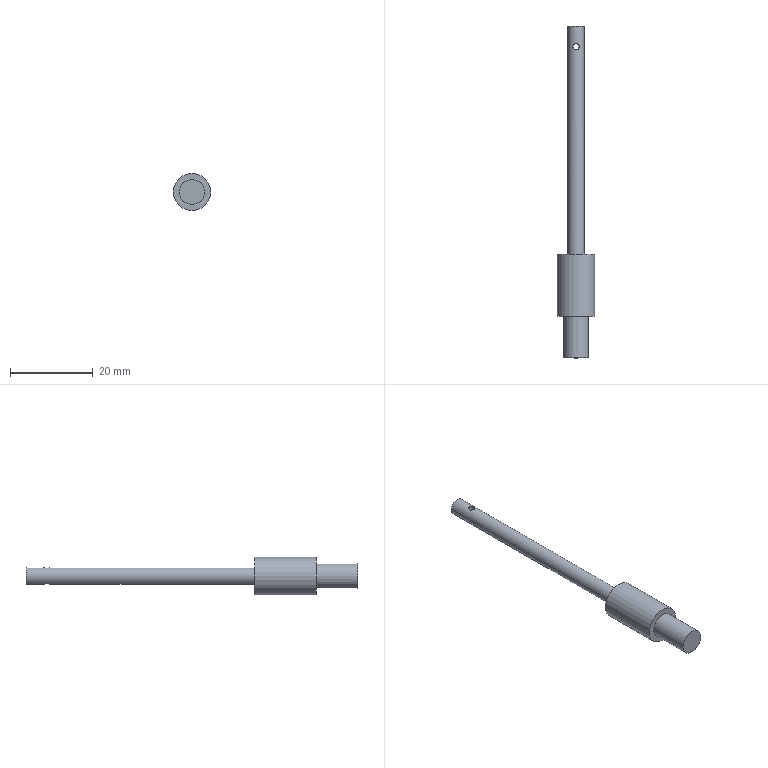Component | NX | PIN | 1 solid | 8 faces | box 9 x 80 x 9 mm | volume 1921 mm3 | cylinder 4 | plane 4 | commonest cylinder face diameters 6 x1 9 x1 4 x1 1.5 x1
STEP:
#1=CARTESIAN_POINT('',(0.,0.,0.));
#2=DIRECTION('',(0.,0.,1.));
#3=DIRECTION('',(1.,0.,0.));
#4=AXIS2_PLACEMENT_3D('',#1,#2,#3);
#5=CARTESIAN_POINT('',(-3.,0.,33.5));
#6=VERTEX_POINT('',#5);
#7=CARTESIAN_POINT('',(0.,0.,33.5));
#8=DIRECTION('',(0.,1.,0.));
#9=DIRECTION('',(-1.,0.,0.));
#10=AXIS2_PLACEMENT_3D('',#7,#8,#9);
#11=CIRCLE('',#10,3.);
#12=CARTESIAN_POINT('',(0.,0.,33.5));
#13=DIRECTION('',(0.,-1.,0.));
#14=DIRECTION('',(0.,0.,1.));
#15=AXIS2_PLACEMENT_3D('',#12,#13,#14);
#16=CYLINDRICAL_SURFACE('',#15,3.);
#17=CARTESIAN_POINT('',(7.854,0.));
#18=DIRECTION('',(-1.,0.));
#19=VECTOR('',#18,1.);
#20=LINE('',#17,#19);
#21=(GEOMETRIC_REPRESENTATION_CONTEXT(2)PARAMETRIC_REPRESENTATION_CONTEXT()REPRESENTATION_CONTEXT('',''));
#22=DEFINITIONAL_REPRESENTATION('',(#20),#21);
#23=PCURVE('',#16,#22);
#24=CARTESIAN_POINT('',(0.,0.,33.5));
#25=DIRECTION('',(0.,1.,0.));
#26=DIRECTION('',(0.,0.,-1.));
#27=AXIS2_PLACEMENT_3D('',#24,#25,#26);
#28=PLANE('',#27);
#29=CARTESIAN_POINT('',(0.,0.));
#30=DIRECTION('',(0.,1.));
#31=AXIS2_PLACEMENT_2D('',#29,#30);
#32=CIRCLE('',#31,3.);
#33=(GEOMETRIC_REPRESENTATION_CONTEXT(2)PARAMETRIC_REPRESENTATION_CONTEXT()REPRESENTATION_CONTEXT('',''));
#34=DEFINITIONAL_REPRESENTATION('',(#32),#33);
#35=PCURVE('',#28,#34);
#36=SURFACE_CURVE('',#11,(#23,#35),.PCURVE_S1.);
#37=EDGE_CURVE('',#6,#6,#36,.T.);
#38=ORIENTED_EDGE('',*,*,#37,.F.);
#39=CARTESIAN_POINT('',(-3.,-10.,33.5));
#40=VERTEX_POINT('',#39);
#41=CARTESIAN_POINT('',(-3.,0.,33.5));
#42=CARTESIAN_POINT('',(-3.,-10.,33.5));
#43=B_SPLINE_CURVE_WITH_KNOTS('',1,(#41,#42),.UNSPECIFIED.,.F.,.F.,(2,2),(0.,10.),.PIECEWISE_BEZIER_KNOTS.);
#44=CARTESIAN_POINT('',(7.854,0.));
#45=DIRECTION('',(0.,1.));
#46=VECTOR('',#45,1.);
#47=LINE('',#44,#46);
#48=(GEOMETRIC_REPRESENTATION_CONTEXT(2)PARAMETRIC_REPRESENTATION_CONTEXT()REPRESENTATION_CONTEXT('',''));
#49=DEFINITIONAL_REPRESENTATION('',(#47),#48);
#50=PCURVE('',#16,#49);
#51=CARTESIAN_POINT('',(1.571,0.));
#52=DIRECTION('',(0.,1.));
#53=VECTOR('',#52,1.);
#54=LINE('',#51,#53);
#55=(GEOMETRIC_REPRESENTATION_CONTEXT(2)PARAMETRIC_REPRESENTATION_CONTEXT()REPRESENTATION_CONTEXT('',''));
#56=DEFINITIONAL_REPRESENTATION('',(#54),#55);
#57=PCURVE('',#16,#56);
#58=SEAM_CURVE('',#43,(#50,#57),.PCURVE_S1.);
#59=EDGE_CURVE('',#6,#40,#58,.T.);
#60=ORIENTED_EDGE('',*,*,#59,.T.);
#61=CARTESIAN_POINT('',(0.,-10.,33.5));
#62=DIRECTION('',(0.,1.,0.));
#63=DIRECTION('',(-1.,0.,0.));
#64=AXIS2_PLACEMENT_3D('',#61,#62,#63);
#65=CIRCLE('',#64,3.);
#66=CARTESIAN_POINT('',(7.854,10.));
#67=DIRECTION('',(-1.,0.));
#68=VECTOR('',#67,1.);
#69=LINE('',#66,#68);
#70=(GEOMETRIC_REPRESENTATION_CONTEXT(2)PARAMETRIC_REPRESENTATION_CONTEXT()REPRESENTATION_CONTEXT('',''));
#71=DEFINITIONAL_REPRESENTATION('',(#69),#70);
#72=PCURVE('',#16,#71);
#73=CARTESIAN_POINT('',(0.,-10.,33.5));
#74=DIRECTION('',(0.,1.,0.));
#75=DIRECTION('',(0.,0.,-1.));
#76=AXIS2_PLACEMENT_3D('',#73,#74,#75);
#77=PLANE('',#76);
#78=CARTESIAN_POINT('',(0.,0.));
#79=DIRECTION('',(0.,1.));
#80=AXIS2_PLACEMENT_2D('',#78,#79);
#81=CIRCLE('',#80,3.);
#82=(GEOMETRIC_REPRESENTATION_CONTEXT(2)PARAMETRIC_REPRESENTATION_CONTEXT()REPRESENTATION_CONTEXT('',''));
#83=DEFINITIONAL_REPRESENTATION('',(#81),#82);
#84=PCURVE('',#77,#83);
#85=SURFACE_CURVE('',#65,(#72,#84),.PCURVE_S1.);
#86=EDGE_CURVE('',#40,#40,#85,.T.);
#87=ORIENTED_EDGE('',*,*,#86,.T.);
#88=ORIENTED_EDGE('',*,*,#59,.F.);
#89=EDGE_LOOP('',(#38,#60,#87,#88));
#90=FACE_BOUND('',#89,.T.);
#91=ADVANCED_FACE('',(#90),#16,.T.);
#92=ORIENTED_EDGE('',*,*,#86,.F.);
#93=EDGE_LOOP('',(#92));
#94=FACE_BOUND('',#93,.T.);
#95=ADVANCED_FACE('',(#94),#77,.F.);
#96=CARTESIAN_POINT('',(-4.5,15.,33.5));
#97=VERTEX_POINT('',#96);
#98=CARTESIAN_POINT('',(0.,15.,33.5));
#99=DIRECTION('',(0.,1.,0.));
#100=DIRECTION('',(-1.,0.,0.));
#101=AXIS2_PLACEMENT_3D('',#98,#99,#100);
#102=CIRCLE('',#101,4.5);
#103=CARTESIAN_POINT('',(0.,15.,33.5));
#104=DIRECTION('',(0.,-1.,0.));
#105=DIRECTION('',(0.,0.,1.));
#106=AXIS2_PLACEMENT_3D('',#103,#104,#105);
#107=CYLINDRICAL_SURFACE('',#106,4.5);
#108=CARTESIAN_POINT('',(7.854,0.));
#109=DIRECTION('',(-1.,0.));
#110=VECTOR('',#109,1.);
#111=LINE('',#108,#110);
#112=(GEOMETRIC_REPRESENTATION_CONTEXT(2)PARAMETRIC_REPRESENTATION_CONTEXT()REPRESENTATION_CONTEXT('',''));
#113=DEFINITIONAL_REPRESENTATION('',(#111),#112);
#114=PCURVE('',#107,#113);
#115=CARTESIAN_POINT('',(0.,15.,33.5));
#116=DIRECTION('',(0.,1.,0.));
#117=DIRECTION('',(0.,0.,-1.));
#118=AXIS2_PLACEMENT_3D('',#115,#116,#117);
#119=PLANE('',#118);
#120=CARTESIAN_POINT('',(0.,0.));
#121=DIRECTION('',(0.,1.));
#122=AXIS2_PLACEMENT_2D('',#120,#121);
#123=CIRCLE('',#122,4.5);
#124=(GEOMETRIC_REPRESENTATION_CONTEXT(2)PARAMETRIC_REPRESENTATION_CONTEXT()REPRESENTATION_CONTEXT('',''));
#125=DEFINITIONAL_REPRESENTATION('',(#123),#124);
#126=PCURVE('',#119,#125);
#127=SURFACE_CURVE('',#102,(#114,#126),.PCURVE_S1.);
#128=EDGE_CURVE('',#97,#97,#127,.T.);
#129=ORIENTED_EDGE('',*,*,#128,.F.);
#130=CARTESIAN_POINT('',(-4.5,0.,33.5));
#131=VERTEX_POINT('',#130);
#132=CARTESIAN_POINT('',(-4.5,15.,33.5));
#133=CARTESIAN_POINT('',(-4.5,0.,33.5));
#134=B_SPLINE_CURVE_WITH_KNOTS('',1,(#132,#133),.UNSPECIFIED.,.F.,.F.,(2,2),(0.,15.),.PIECEWISE_BEZIER_KNOTS.);
#135=CARTESIAN_POINT('',(7.854,0.));
#136=DIRECTION('',(0.,1.));
#137=VECTOR('',#136,1.);
#138=LINE('',#135,#137);
#139=(GEOMETRIC_REPRESENTATION_CONTEXT(2)PARAMETRIC_REPRESENTATION_CONTEXT()REPRESENTATION_CONTEXT('',''));
#140=DEFINITIONAL_REPRESENTATION('',(#138),#139);
#141=PCURVE('',#107,#140);
#142=CARTESIAN_POINT('',(1.571,0.));
#143=DIRECTION('',(0.,1.));
#144=VECTOR('',#143,1.);
#145=LINE('',#142,#144);
#146=(GEOMETRIC_REPRESENTATION_CONTEXT(2)PARAMETRIC_REPRESENTATION_CONTEXT()REPRESENTATION_CONTEXT('',''));
#147=DEFINITIONAL_REPRESENTATION('',(#145),#146);
#148=PCURVE('',#107,#147);
#149=SEAM_CURVE('',#134,(#141,#148),.PCURVE_S1.);
#150=EDGE_CURVE('',#97,#131,#149,.T.);
#151=ORIENTED_EDGE('',*,*,#150,.T.);
#152=CARTESIAN_POINT('',(0.,0.,33.5));
#153=DIRECTION('',(0.,1.,0.));
#154=DIRECTION('',(-1.,0.,0.));
#155=AXIS2_PLACEMENT_3D('',#152,#153,#154);
#156=CIRCLE('',#155,4.5);
#157=CARTESIAN_POINT('',(7.854,15.));
#158=DIRECTION('',(-1.,0.));
#159=VECTOR('',#158,1.);
#160=LINE('',#157,#159);
#161=(GEOMETRIC_REPRESENTATION_CONTEXT(2)PARAMETRIC_REPRESENTATION_CONTEXT()REPRESENTATION_CONTEXT('',''));
#162=DEFINITIONAL_REPRESENTATION('',(#160),#161);
#163=PCURVE('',#107,#162);
#164=CARTESIAN_POINT('',(0.,0.));
#165=DIRECTION('',(0.,1.));
#166=AXIS2_PLACEMENT_2D('',#164,#165);
#167=CIRCLE('',#166,4.5);
#168=(GEOMETRIC_REPRESENTATION_CONTEXT(2)PARAMETRIC_REPRESENTATION_CONTEXT()REPRESENTATION_CONTEXT('',''));
#169=DEFINITIONAL_REPRESENTATION('',(#167),#168);
#170=PCURVE('',#28,#169);
#171=SURFACE_CURVE('',#156,(#163,#170),.PCURVE_S1.);
#172=EDGE_CURVE('',#131,#131,#171,.T.);
#173=ORIENTED_EDGE('',*,*,#172,.T.);
#174=ORIENTED_EDGE('',*,*,#150,.F.);
#175=EDGE_LOOP('',(#129,#151,#173,#174));
#176=FACE_BOUND('',#175,.T.);
#177=ADVANCED_FACE('',(#176),#107,.T.);
#178=CARTESIAN_POINT('',(-2.,15.,33.5));
#179=VERTEX_POINT('',#178);
#180=CARTESIAN_POINT('',(0.,15.,33.5));
#181=DIRECTION('',(0.,1.,0.));
#182=DIRECTION('',(-1.,0.,0.));
#183=AXIS2_PLACEMENT_3D('',#180,#181,#182);
#184=CIRCLE('',#183,2.);
#185=CARTESIAN_POINT('',(0.,0.));
#186=DIRECTION('',(0.,1.));
#187=AXIS2_PLACEMENT_2D('',#185,#186);
#188=CIRCLE('',#187,2.);
#189=(GEOMETRIC_REPRESENTATION_CONTEXT(2)PARAMETRIC_REPRESENTATION_CONTEXT()REPRESENTATION_CONTEXT('',''));
#190=DEFINITIONAL_REPRESENTATION('',(#188),#189);
#191=PCURVE('',#119,#190);
#192=CARTESIAN_POINT('',(0.,70.,33.5));
#193=DIRECTION('',(0.,-1.,0.));
#194=DIRECTION('',(0.,0.,1.));
#195=AXIS2_PLACEMENT_3D('',#192,#193,#194);
#196=CYLINDRICAL_SURFACE('',#195,2.);
#197=CARTESIAN_POINT('',(7.854,55.));
#198=DIRECTION('',(-1.,0.));
#199=VECTOR('',#198,1.);
#200=LINE('',#197,#199);
#201=(GEOMETRIC_REPRESENTATION_CONTEXT(2)PARAMETRIC_REPRESENTATION_CONTEXT()REPRESENTATION_CONTEXT('',''));
#202=DEFINITIONAL_REPRESENTATION('',(#200),#201);
#203=PCURVE('',#196,#202);
#204=SURFACE_CURVE('',#184,(#191,#203),.PCURVE_S1.);
#205=EDGE_CURVE('',#179,#179,#204,.T.);
#206=ORIENTED_EDGE('',*,*,#205,.F.);
#207=EDGE_LOOP('',(#206));
#208=FACE_BOUND('',#207,.T.);
#209=ORIENTED_EDGE('',*,*,#128,.T.);
#210=EDGE_LOOP('',(#209));
#211=FACE_BOUND('',#210,.T.);
#212=ADVANCED_FACE('',(#208,#211),#119,.T.);
#213=ORIENTED_EDGE('',*,*,#37,.T.);
#214=EDGE_LOOP('',(#213));
#215=FACE_BOUND('',#214,.T.);
#216=ORIENTED_EDGE('',*,*,#172,.F.);
#217=EDGE_LOOP('',(#216));
#218=FACE_BOUND('',#217,.T.);
#219=ADVANCED_FACE('',(#215,#218),#28,.F.);
#220=CARTESIAN_POINT('',(-2.,70.,33.5));
#221=VERTEX_POINT('',#220);
#222=CARTESIAN_POINT('',(0.,70.,33.5));
#223=DIRECTION('',(0.,1.,0.));
#224=DIRECTION('',(-1.,0.,0.));
#225=AXIS2_PLACEMENT_3D('',#222,#223,#224);
#226=CIRCLE('',#225,2.);
#227=CARTESIAN_POINT('',(7.854,0.));
#228=DIRECTION('',(-1.,0.));
#229=VECTOR('',#228,1.);
#230=LINE('',#227,#229);
#231=(GEOMETRIC_REPRESENTATION_CONTEXT(2)PARAMETRIC_REPRESENTATION_CONTEXT()REPRESENTATION_CONTEXT('',''));
#232=DEFINITIONAL_REPRESENTATION('',(#230),#231);
#233=PCURVE('',#196,#232);
#234=CARTESIAN_POINT('',(0.,70.,33.5));
#235=DIRECTION('',(0.,1.,0.));
#236=DIRECTION('',(0.,0.,-1.));
#237=AXIS2_PLACEMENT_3D('',#234,#235,#236);
#238=PLANE('',#237);
#239=CARTESIAN_POINT('',(0.,0.));
#240=DIRECTION('',(0.,1.));
#241=AXIS2_PLACEMENT_2D('',#239,#240);
#242=CIRCLE('',#241,2.);
#243=(GEOMETRIC_REPRESENTATION_CONTEXT(2)PARAMETRIC_REPRESENTATION_CONTEXT()REPRESENTATION_CONTEXT('',''));
#244=DEFINITIONAL_REPRESENTATION('',(#242),#243);
#245=PCURVE('',#238,#244);
#246=SURFACE_CURVE('',#226,(#233,#245),.PCURVE_S1.);
#247=EDGE_CURVE('',#221,#221,#246,.T.);
#248=ORIENTED_EDGE('',*,*,#247,.F.);
#249=CARTESIAN_POINT('',(-2.,70.,33.5));
#250=CARTESIAN_POINT('',(-2.,15.,33.5));
#251=B_SPLINE_CURVE_WITH_KNOTS('',1,(#249,#250),.UNSPECIFIED.,.F.,.F.,(2,2),(0.,55.),.PIECEWISE_BEZIER_KNOTS.);
#252=CARTESIAN_POINT('',(7.854,0.));
#253=DIRECTION('',(0.,1.));
#254=VECTOR('',#253,1.);
#255=LINE('',#252,#254);
#256=(GEOMETRIC_REPRESENTATION_CONTEXT(2)PARAMETRIC_REPRESENTATION_CONTEXT()REPRESENTATION_CONTEXT('',''));
#257=DEFINITIONAL_REPRESENTATION('',(#255),#256);
#258=PCURVE('',#196,#257);
#259=CARTESIAN_POINT('',(1.571,0.));
#260=DIRECTION('',(0.,1.));
#261=VECTOR('',#260,1.);
#262=LINE('',#259,#261);
#263=(GEOMETRIC_REPRESENTATION_CONTEXT(2)PARAMETRIC_REPRESENTATION_CONTEXT()REPRESENTATION_CONTEXT('',''));
#264=DEFINITIONAL_REPRESENTATION('',(#262),#263);
#265=PCURVE('',#196,#264);
#266=SEAM_CURVE('',#251,(#258,#265),.PCURVE_S1.);
#267=EDGE_CURVE('',#221,#179,#266,.T.);
#268=ORIENTED_EDGE('',*,*,#267,.T.);
#269=ORIENTED_EDGE('',*,*,#205,.T.);
#270=ORIENTED_EDGE('',*,*,#267,.F.);
#271=EDGE_LOOP('',(#248,#268,#269,#270));
#272=FACE_BOUND('',#271,.T.);
#273=CARTESIAN_POINT('',(0.,65.75,35.5));
#274=VERTEX_POINT('',#273);
#275=CARTESIAN_POINT('',(0.,65.75,35.5));
#276=CARTESIAN_POINT('',(0.08082,65.75,35.5));
#277=CARTESIAN_POINT('',(0.1627,65.737,35.495));
#278=CARTESIAN_POINT('',(0.2389,65.711,35.486));
#279=CARTESIAN_POINT('',(0.3149,65.685,35.477));
#280=CARTESIAN_POINT('',(0.3872,65.647,35.463));
#281=CARTESIAN_POINT('',(0.4506,65.6,35.449));
#282=CARTESIAN_POINT('',(0.5165,65.55,35.433));
#283=CARTESIAN_POINT('',(0.5746,65.489,35.416));
#284=CARTESIAN_POINT('',(0.6209,65.421,35.401));
#285=CARTESIAN_POINT('',(0.6689,65.35,35.386));
#286=CARTESIAN_POINT('',(0.7053,65.269,35.372));
#287=CARTESIAN_POINT('',(0.7267,65.185,35.363));
#288=CARTESIAN_POINT('',(0.7472,65.105,35.355));
#289=CARTESIAN_POINT('',(0.7544,65.019,35.352));
#290=CARTESIAN_POINT('',(0.7473,64.936,35.355));
#291=CARTESIAN_POINT('',(0.7406,64.858,35.358));
#292=CARTESIAN_POINT('',(0.7213,64.78,35.366));
#293=CARTESIAN_POINT('',(0.6912,64.709,35.377));
#294=CARTESIAN_POINT('',(0.6605,64.636,35.388));
#295=CARTESIAN_POINT('',(0.6179,64.568,35.403));
#296=CARTESIAN_POINT('',(0.5665,64.508,35.418));
#297=CARTESIAN_POINT('',(0.5116,64.445,35.434));
#298=CARTESIAN_POINT('',(0.4452,64.391,35.451));
#299=CARTESIAN_POINT('',(0.3721,64.349,35.465));
#300=CARTESIAN_POINT('',(0.298,64.306,35.479));
#301=CARTESIAN_POINT('',(0.2147,64.276,35.49));
#302=CARTESIAN_POINT('',(0.1297,64.261,35.496));
#303=CARTESIAN_POINT('',(0.04914,64.247,35.501));
#304=CARTESIAN_POINT('',(-0.03529,64.246,35.501));
#305=CARTESIAN_POINT('',(-0.1161,64.259,35.497));
#306=CARTESIAN_POINT('',(-0.1938,64.271,35.492));
#307=CARTESIAN_POINT('',(-0.2703,64.296,35.483));
#308=CARTESIAN_POINT('',(-0.3397,64.331,35.471));
#309=CARTESIAN_POINT('',(-0.4112,64.368,35.459));
#310=CARTESIAN_POINT('',(-0.4772,64.416,35.443));
#311=CARTESIAN_POINT('',(-0.5332,64.473,35.428));
#312=CARTESIAN_POINT('',(-0.5925,64.533,35.411));
#313=CARTESIAN_POINT('',(-0.6423,64.604,35.394));
#314=CARTESIAN_POINT('',(-0.6784,64.68,35.381));
#315=CARTESIAN_POINT('',(-0.7147,64.757,35.368));
#316=CARTESIAN_POINT('',(-0.7383,64.843,35.359));
#317=CARTESIAN_POINT('',(-0.7466,64.928,35.355));
#318=CARTESIAN_POINT('',(-0.7543,65.008,35.352));
#319=CARTESIAN_POINT('',(-0.7488,65.091,35.355));
#320=CARTESIAN_POINT('',(-0.7306,65.169,35.362));
#321=CARTESIAN_POINT('',(-0.713,65.245,35.369));
#322=CARTESIAN_POINT('',(-0.6832,65.319,35.38));
#323=CARTESIAN_POINT('',(-0.6437,65.385,35.394));
#324=CARTESIAN_POINT('',(-0.602,65.455,35.408));
#325=CARTESIAN_POINT('',(-0.5486,65.518,35.424));
#326=CARTESIAN_POINT('',(-0.4871,65.57,35.44));
#327=CARTESIAN_POINT('',(-0.4223,65.626,35.456));
#328=CARTESIAN_POINT('',(-0.3467,65.671,35.471));
#329=CARTESIAN_POINT('',(-0.2662,65.701,35.482));
#330=CARTESIAN_POINT('',(-0.1823,65.733,35.493));
#331=CARTESIAN_POINT('',(-0.09041,65.75,35.5));
#332=CARTESIAN_POINT('',(0.,65.75,35.5));
#333=B_SPLINE_CURVE_WITH_KNOTS('',3,(#275,#276,#277,#278,#279,#280,#281,#282,#283,#284,#285,#286,#287,#288,#289,#290,#291,#292,#293,#294,#295,#296,#297,#298,#299,#300,#301,#302,#303,#304,#305,#306,#307,#308,#309,#310,#311,#312,#313,#314,#315,#316,#317,#318,#319,#320,#321,#322,#323,#324,#325,#326,#327,#328,#329,#330,#331,#332),.UNSPECIFIED.,.T.,.F.,(1,3,3,3,3,3,3,3,3,3,3,3,3,3,3,3,3,3,3,3,3,1),(-0.05748,0.,0.05123,0.1023,0.1554,0.2106,0.2635,0.3131,0.3637,0.4177,0.4726,0.5246,0.5744,0.6258,0.6802,0.7349,0.786,0.8354,0.8875,0.9425,1.,1.051),.UNSPECIFIED.);
#334=CARTESIAN_POINT('',(6.283,4.25));
#335=CARTESIAN_POINT('',(6.274,4.25));
#336=CARTESIAN_POINT('',(6.256,4.251));
#337=CARTESIAN_POINT('',(6.229,4.257));
#338=CARTESIAN_POINT('',(6.203,4.267));
#339=CARTESIAN_POINT('',(6.176,4.28));
#340=CARTESIAN_POINT('',(6.151,4.297));
#341=CARTESIAN_POINT('',(6.126,4.318));
#342=CARTESIAN_POINT('',(6.102,4.342));
#343=CARTESIAN_POINT('',(6.078,4.369));
#344=CARTESIAN_POINT('',(6.056,4.4));
#345=CARTESIAN_POINT('',(6.035,4.433));
#346=CARTESIAN_POINT('',(6.015,4.469));
#347=CARTESIAN_POINT('',(5.996,4.508));
#348=CARTESIAN_POINT('',(5.978,4.55));
#349=CARTESIAN_POINT('',(5.962,4.593));
#350=CARTESIAN_POINT('',(5.948,4.639));
#351=CARTESIAN_POINT('',(5.935,4.687));
#352=CARTESIAN_POINT('',(5.924,4.736));
#353=CARTESIAN_POINT('',(5.915,4.787));
#354=CARTESIAN_POINT('',(5.908,4.839));
#355=CARTESIAN_POINT('',(5.903,4.892));
#356=CARTESIAN_POINT('',(5.9,4.946));
#357=CARTESIAN_POINT('',(5.898,5.));
#358=CARTESIAN_POINT('',(5.899,5.054));
#359=CARTESIAN_POINT('',(5.903,5.107));
#360=CARTESIAN_POINT('',(5.908,5.161));
#361=CARTESIAN_POINT('',(5.915,5.213));
#362=CARTESIAN_POINT('',(5.924,5.264));
#363=CARTESIAN_POINT('',(5.935,5.313));
#364=CARTESIAN_POINT('',(5.948,5.361));
#365=CARTESIAN_POINT('',(5.962,5.407));
#366=CARTESIAN_POINT('',(5.978,5.451));
#367=CARTESIAN_POINT('',(5.996,5.492));
#368=CARTESIAN_POINT('',(6.015,5.531));
#369=CARTESIAN_POINT('',(6.035,5.567));
#370=CARTESIAN_POINT('',(6.056,5.6));
#371=CARTESIAN_POINT('',(6.078,5.631));
#372=CARTESIAN_POINT('',(6.102,5.658));
#373=CARTESIAN_POINT('',(6.126,5.682));
#374=CARTESIAN_POINT('',(6.151,5.703));
#375=CARTESIAN_POINT('',(6.176,5.72));
#376=CARTESIAN_POINT('',(6.203,5.733));
#377=CARTESIAN_POINT('',(6.229,5.743));
#378=CARTESIAN_POINT('',(6.256,5.749));
#379=CARTESIAN_POINT('',(6.283,5.751));
#380=CARTESIAN_POINT('',(6.31,5.749));
#381=CARTESIAN_POINT('',(6.337,5.743));
#382=CARTESIAN_POINT('',(6.364,5.733));
#383=CARTESIAN_POINT('',(6.39,5.72));
#384=CARTESIAN_POINT('',(6.416,5.703));
#385=CARTESIAN_POINT('',(6.441,5.682));
#386=CARTESIAN_POINT('',(6.465,5.658));
#387=CARTESIAN_POINT('',(6.488,5.631));
#388=CARTESIAN_POINT('',(6.511,5.6));
#389=CARTESIAN_POINT('',(6.532,5.567));
#390=CARTESIAN_POINT('',(6.552,5.53));
#391=CARTESIAN_POINT('',(6.571,5.492));
#392=CARTESIAN_POINT('',(6.588,5.45));
#393=CARTESIAN_POINT('',(6.604,5.407));
#394=CARTESIAN_POINT('',(6.619,5.361));
#395=CARTESIAN_POINT('',(6.631,5.313));
#396=CARTESIAN_POINT('',(6.642,5.264));
#397=CARTESIAN_POINT('',(6.651,5.213));
#398=CARTESIAN_POINT('',(6.659,5.161));
#399=CARTESIAN_POINT('',(6.664,5.108));
#400=CARTESIAN_POINT('',(6.667,5.054));
#401=CARTESIAN_POINT('',(6.668,5.));
#402=CARTESIAN_POINT('',(6.667,4.946));
#403=CARTESIAN_POINT('',(6.664,4.892));
#404=CARTESIAN_POINT('',(6.659,4.839));
#405=CARTESIAN_POINT('',(6.651,4.787));
#406=CARTESIAN_POINT('',(6.642,4.736));
#407=CARTESIAN_POINT('',(6.631,4.686));
#408=CARTESIAN_POINT('',(6.618,4.639));
#409=CARTESIAN_POINT('',(6.604,4.593));
#410=CARTESIAN_POINT('',(6.588,4.549));
#411=CARTESIAN_POINT('',(6.57,4.508));
#412=CARTESIAN_POINT('',(6.552,4.469));
#413=CARTESIAN_POINT('',(6.532,4.433));
#414=CARTESIAN_POINT('',(6.51,4.4));
#415=CARTESIAN_POINT('',(6.488,4.369));
#416=CARTESIAN_POINT('',(6.464,4.342));
#417=CARTESIAN_POINT('',(6.44,4.318));
#418=CARTESIAN_POINT('',(6.415,4.297));
#419=CARTESIAN_POINT('',(6.39,4.28));
#420=CARTESIAN_POINT('',(6.364,4.267));
#421=CARTESIAN_POINT('',(6.337,4.257));
#422=CARTESIAN_POINT('',(6.31,4.251));
#423=CARTESIAN_POINT('',(6.292,4.25));
#424=CARTESIAN_POINT('',(6.283,4.25));
#425=B_SPLINE_CURVE_WITH_KNOTS('',3,(#334,#335,#336,#337,#338,#339,#340,#341,#342,#343,#344,#345,#346,#347,#348,#349,#350,#351,#352,#353,#354,#355,#356,#357,#358,#359,#360,#361,#362,#363,#364,#365,#366,#367,#368,#369,#370,#371,#372,#373,#374,#375,#376,#377,#378,#379,#380,#381,#382,#383,#384,#385,#386,#387,#388,#389,#390,#391,#392,#393,#394,#395,#396,#397,#398,#399,#400,#401,#402,#403,#404,#405,#406,#407,#408,#409,#410,#411,#412,#413,#414,#415,#416,#417,#418,#419,#420,#421,#422,#423,#424),.UNSPECIFIED.,.T.,.F.,(4,1,1,1,1,1,1,1,1,1,1,1,1,1,1,1,1,1,1,1,1,1,1,1,1,1,1,1,1,1,1,1,1,1,1,1,1,1,1,1,1,1,1,1,1,1,1,1,1,1,1,1,1,1,1,1,1,1,1,1,1,1,1,1,1,1,1,1,1,1,1,1,1,1,1,1,1,1,1,1,1,1,1,1,1,1,1,1,4),(0.,0.01136,0.02273,0.03409,0.04545,0.05682,0.06818,0.07955,0.09091,0.1023,0.1136,0.125,0.1364,0.1477,0.1591,0.1705,0.1818,0.1932,0.2045,0.2159,0.2273,0.2386,0.25,0.2614,0.2727,0.2841,0.2955,0.3068,0.3182,0.3295,0.3409,0.3523,0.3636,0.375,0.3864,0.3977,0.4091,0.4205,0.4318,0.4432,0.4545,0.4659,0.4773,0.4886,0.5,0.5114,0.5227,0.5341,0.5455,0.5568,0.5682,0.5795,0.5909,0.6023,0.6136,0.625,0.6364,0.6477,0.6591,0.6705,0.6818,0.6932,0.7045,0.7159,0.7273,0.7386,0.75,0.7614,0.7727,0.7841,0.7955,0.8068,0.8182,0.8295,0.8409,0.8523,0.8636,0.875,0.8864,0.8977,0.9091,0.9205,0.9318,0.9432,0.9545,0.9659,0.9773,0.9886,1.),.QUASI_UNIFORM_KNOTS.);
#426=(GEOMETRIC_REPRESENTATION_CONTEXT(2)PARAMETRIC_REPRESENTATION_CONTEXT()REPRESENTATION_CONTEXT('',''));
#427=DEFINITIONAL_REPRESENTATION('',(#425),#426);
#428=PCURVE('',#196,#427);
#429=CARTESIAN_POINT('',(0.,65.,15.5));
#430=DIRECTION('',(0.,0.,1.));
#431=DIRECTION('',(0.,1.,0.));
#432=AXIS2_PLACEMENT_3D('',#429,#430,#431);
#433=CYLINDRICAL_SURFACE('',#432,0.75);
#434=CARTESIAN_POINT('',(6.283,20.));
#435=CARTESIAN_POINT('',(6.259,20.));
#436=CARTESIAN_POINT('',(6.211,19.999));
#437=CARTESIAN_POINT('',(6.139,19.997));
#438=CARTESIAN_POINT('',(6.067,19.994));
#439=CARTESIAN_POINT('',(5.995,19.989));
#440=CARTESIAN_POINT('',(5.924,19.983));
#441=CARTESIAN_POINT('',(5.852,19.975));
#442=CARTESIAN_POINT('',(5.781,19.967));
#443=CARTESIAN_POINT('',(5.71,19.958));
#444=CARTESIAN_POINT('',(5.639,19.949));
#445=CARTESIAN_POINT('',(5.568,19.939));
#446=CARTESIAN_POINT('',(5.497,19.928));
#447=CARTESIAN_POINT('',(5.427,19.918));
#448=CARTESIAN_POINT('',(5.356,19.908));
#449=CARTESIAN_POINT('',(5.285,19.898));
#450=CARTESIAN_POINT('',(5.214,19.889));
#451=CARTESIAN_POINT('',(5.143,19.88));
#452=CARTESIAN_POINT('',(5.072,19.873));
#453=CARTESIAN_POINT('',(5.,19.866));
#454=CARTESIAN_POINT('',(4.929,19.861));
#455=CARTESIAN_POINT('',(4.857,19.857));
#456=CARTESIAN_POINT('',(4.785,19.855));
#457=CARTESIAN_POINT('',(4.713,19.854));
#458=CARTESIAN_POINT('',(4.641,19.855));
#459=CARTESIAN_POINT('',(4.569,19.857));
#460=CARTESIAN_POINT('',(4.497,19.861));
#461=CARTESIAN_POINT('',(4.425,19.866));
#462=CARTESIAN_POINT('',(4.353,19.873));
#463=CARTESIAN_POINT('',(4.282,19.88));
#464=CARTESIAN_POINT('',(4.211,19.889));
#465=CARTESIAN_POINT('',(4.14,19.898));
#466=CARTESIAN_POINT('',(4.069,19.908));
#467=CARTESIAN_POINT('',(3.998,19.918));
#468=CARTESIAN_POINT('',(3.927,19.928));
#469=CARTESIAN_POINT('',(3.856,19.939));
#470=CARTESIAN_POINT('',(3.785,19.949));
#471=CARTESIAN_POINT('',(3.714,19.958));
#472=CARTESIAN_POINT('',(3.644,19.967));
#473=CARTESIAN_POINT('',(3.573,19.975));
#474=CARTESIAN_POINT('',(3.501,19.983));
#475=CARTESIAN_POINT('',(3.429,19.989));
#476=CARTESIAN_POINT('',(3.358,19.994));
#477=CARTESIAN_POINT('',(3.286,19.997));
#478=CARTESIAN_POINT('',(3.214,19.999));
#479=CARTESIAN_POINT('',(3.142,20.));
#480=CARTESIAN_POINT('',(3.07,19.999));
#481=CARTESIAN_POINT('',(2.998,19.997));
#482=CARTESIAN_POINT('',(2.926,19.994));
#483=CARTESIAN_POINT('',(2.854,19.989));
#484=CARTESIAN_POINT('',(2.782,19.983));
#485=CARTESIAN_POINT('',(2.711,19.975));
#486=CARTESIAN_POINT('',(2.64,19.967));
#487=CARTESIAN_POINT('',(2.569,19.958));
#488=CARTESIAN_POINT('',(2.497,19.949));
#489=CARTESIAN_POINT('',(2.426,19.939));
#490=CARTESIAN_POINT('',(2.356,19.928));
#491=CARTESIAN_POINT('',(2.285,19.918));
#492=CARTESIAN_POINT('',(2.214,19.908));
#493=CARTESIAN_POINT('',(2.143,19.898));
#494=CARTESIAN_POINT('',(2.072,19.889));
#495=CARTESIAN_POINT('',(2.001,19.88));
#496=CARTESIAN_POINT('',(1.93,19.873));
#497=CARTESIAN_POINT('',(1.858,19.866));
#498=CARTESIAN_POINT('',(1.787,19.861));
#499=CARTESIAN_POINT('',(1.715,19.857));
#500=CARTESIAN_POINT('',(1.643,19.855));
#501=CARTESIAN_POINT('',(1.571,19.854));
#502=CARTESIAN_POINT('',(1.499,19.855));
#503=CARTESIAN_POINT('',(1.426,19.857));
#504=CARTESIAN_POINT('',(1.355,19.861));
#505=CARTESIAN_POINT('',(1.283,19.866));
#506=CARTESIAN_POINT('',(1.211,19.873));
#507=CARTESIAN_POINT('',(1.14,19.88));
#508=CARTESIAN_POINT('',(1.068,19.889));
#509=CARTESIAN_POINT('',(0.9977,19.898));
#510=CARTESIAN_POINT('',(0.9267,19.908));
#511=CARTESIAN_POINT('',(0.8557,19.918));
#512=CARTESIAN_POINT('',(0.7848,19.929));
#513=CARTESIAN_POINT('',(0.714,19.939));
#514=CARTESIAN_POINT('',(0.6435,19.949));
#515=CARTESIAN_POINT('',(0.5725,19.958));
#516=CARTESIAN_POINT('',(0.5012,19.967));
#517=CARTESIAN_POINT('',(0.4299,19.976));
#518=CARTESIAN_POINT('',(0.3587,19.983));
#519=CARTESIAN_POINT('',(0.2875,19.989));
#520=CARTESIAN_POINT('',(0.2157,19.994));
#521=CARTESIAN_POINT('',(0.1437,19.997));
#522=CARTESIAN_POINT('',(0.07165,19.999));
#523=CARTESIAN_POINT('',(0.02383,20.));
#524=CARTESIAN_POINT('',(-0.,20.));
#525=B_SPLINE_CURVE_WITH_KNOTS('',3,(#434,#435,#436,#437,#438,#439,#440,#441,#442,#443,#444,#445,#446,#447,#448,#449,#450,#451,#452,#453,#454,#455,#456,#457,#458,#459,#460,#461,#462,#463,#464,#465,#466,#467,#468,#469,#470,#471,#472,#473,#474,#475,#476,#477,#478,#479,#480,#481,#482,#483,#484,#485,#486,#487,#488,#489,#490,#491,#492,#493,#494,#495,#496,#497,#498,#499,#500,#501,#502,#503,#504,#505,#506,#507,#508,#509,#510,#511,#512,#513,#514,#515,#516,#517,#518,#519,#520,#521,#522,#523,#524),.UNSPECIFIED.,.F.,.F.,(4,1,1,1,1,1,1,1,1,1,1,1,1,1,1,1,1,1,1,1,1,1,1,1,1,1,1,1,1,1,1,1,1,1,1,1,1,1,1,1,1,1,1,1,1,1,1,1,1,1,1,1,1,1,1,1,1,1,1,1,1,1,1,1,1,1,1,1,1,1,1,1,1,1,1,1,1,1,1,1,1,1,1,1,1,1,1,1,4),(0.,0.01136,0.02273,0.03409,0.04545,0.05682,0.06818,0.07955,0.09091,0.1023,0.1136,0.125,0.1364,0.1477,0.1591,0.1705,0.1818,0.1932,0.2045,0.2159,0.2273,0.2386,0.25,0.2614,0.2727,0.2841,0.2955,0.3068,0.3182,0.3295,0.3409,0.3523,0.3636,0.375,0.3864,0.3977,0.4091,0.4205,0.4318,0.4432,0.4545,0.4659,0.4773,0.4886,0.5,0.5114,0.5227,0.5341,0.5455,0.5568,0.5682,0.5795,0.5909,0.6023,0.6136,0.625,0.6364,0.6477,0.6591,0.6705,0.6818,0.6932,0.7045,0.7159,0.7273,0.7386,0.75,0.7614,0.7727,0.7841,0.7955,0.8068,0.8182,0.8295,0.8409,0.8523,0.8636,0.875,0.8864,0.8977,0.9091,0.9205,0.9318,0.9432,0.9545,0.9659,0.9773,0.9886,1.),.QUASI_UNIFORM_KNOTS.);
#526=(GEOMETRIC_REPRESENTATION_CONTEXT(2)PARAMETRIC_REPRESENTATION_CONTEXT()REPRESENTATION_CONTEXT('',''));
#527=DEFINITIONAL_REPRESENTATION('',(#525),#526);
#528=PCURVE('',#433,#527);
#529=SURFACE_CURVE('',#333,(#428,#528),.PCURVE_S1.);
#530=EDGE_CURVE('',#274,#274,#529,.T.);
#531=ORIENTED_EDGE('',*,*,#530,.T.);
#532=EDGE_LOOP('',(#531));
#533=FACE_BOUND('',#532,.T.);
#534=CARTESIAN_POINT('',(0.,65.75,31.5));
#535=VERTEX_POINT('',#534);
#536=CARTESIAN_POINT('',(0.,65.75,31.5));
#537=CARTESIAN_POINT('',(-0.08082,65.75,31.5));
#538=CARTESIAN_POINT('',(-0.1627,65.737,31.505));
#539=CARTESIAN_POINT('',(-0.2389,65.711,31.514));
#540=CARTESIAN_POINT('',(-0.3149,65.685,31.523));
#541=CARTESIAN_POINT('',(-0.3872,65.647,31.537));
#542=CARTESIAN_POINT('',(-0.4506,65.6,31.551));
#543=CARTESIAN_POINT('',(-0.5165,65.55,31.567));
#544=CARTESIAN_POINT('',(-0.5746,65.489,31.584));
#545=CARTESIAN_POINT('',(-0.6209,65.421,31.599));
#546=CARTESIAN_POINT('',(-0.6689,65.35,31.614));
#547=CARTESIAN_POINT('',(-0.7053,65.269,31.628));
#548=CARTESIAN_POINT('',(-0.7267,65.185,31.637));
#549=CARTESIAN_POINT('',(-0.7472,65.105,31.645));
#550=CARTESIAN_POINT('',(-0.7544,65.019,31.648));
#551=CARTESIAN_POINT('',(-0.7473,64.936,31.645));
#552=CARTESIAN_POINT('',(-0.7406,64.858,31.642));
#553=CARTESIAN_POINT('',(-0.7213,64.78,31.634));
#554=CARTESIAN_POINT('',(-0.6912,64.709,31.623));
#555=CARTESIAN_POINT('',(-0.6605,64.636,31.612));
#556=CARTESIAN_POINT('',(-0.6179,64.568,31.597));
#557=CARTESIAN_POINT('',(-0.5665,64.508,31.582));
#558=CARTESIAN_POINT('',(-0.5116,64.445,31.566));
#559=CARTESIAN_POINT('',(-0.4452,64.391,31.549));
#560=CARTESIAN_POINT('',(-0.3721,64.349,31.535));
#561=CARTESIAN_POINT('',(-0.298,64.306,31.521));
#562=CARTESIAN_POINT('',(-0.2147,64.276,31.51));
#563=CARTESIAN_POINT('',(-0.1297,64.261,31.504));
#564=CARTESIAN_POINT('',(-0.04914,64.247,31.499));
#565=CARTESIAN_POINT('',(0.03529,64.246,31.499));
#566=CARTESIAN_POINT('',(0.1161,64.259,31.503));
#567=CARTESIAN_POINT('',(0.1938,64.271,31.508));
#568=CARTESIAN_POINT('',(0.2703,64.296,31.517));
#569=CARTESIAN_POINT('',(0.3397,64.331,31.529));
#570=CARTESIAN_POINT('',(0.4112,64.368,31.541));
#571=CARTESIAN_POINT('',(0.4772,64.416,31.557));
#572=CARTESIAN_POINT('',(0.5332,64.473,31.572));
#573=CARTESIAN_POINT('',(0.5925,64.533,31.589));
#574=CARTESIAN_POINT('',(0.6423,64.604,31.606));
#575=CARTESIAN_POINT('',(0.6784,64.68,31.619));
#576=CARTESIAN_POINT('',(0.7147,64.757,31.632));
#577=CARTESIAN_POINT('',(0.7383,64.843,31.641));
#578=CARTESIAN_POINT('',(0.7466,64.928,31.645));
#579=CARTESIAN_POINT('',(0.7543,65.008,31.648));
#580=CARTESIAN_POINT('',(0.7488,65.091,31.645));
#581=CARTESIAN_POINT('',(0.7306,65.169,31.638));
#582=CARTESIAN_POINT('',(0.713,65.245,31.631));
#583=CARTESIAN_POINT('',(0.6832,65.319,31.62));
#584=CARTESIAN_POINT('',(0.6437,65.385,31.606));
#585=CARTESIAN_POINT('',(0.602,65.455,31.592));
#586=CARTESIAN_POINT('',(0.5486,65.518,31.576));
#587=CARTESIAN_POINT('',(0.4871,65.57,31.56));
#588=CARTESIAN_POINT('',(0.4223,65.626,31.544));
#589=CARTESIAN_POINT('',(0.3467,65.671,31.529));
#590=CARTESIAN_POINT('',(0.2662,65.701,31.518));
#591=CARTESIAN_POINT('',(0.1823,65.733,31.507));
#592=CARTESIAN_POINT('',(0.09041,65.75,31.5));
#593=CARTESIAN_POINT('',(0.,65.75,31.5));
#594=B_SPLINE_CURVE_WITH_KNOTS('',3,(#536,#537,#538,#539,#540,#541,#542,#543,#544,#545,#546,#547,#548,#549,#550,#551,#552,#553,#554,#555,#556,#557,#558,#559,#560,#561,#562,#563,#564,#565,#566,#567,#568,#569,#570,#571,#572,#573,#574,#575,#576,#577,#578,#579,#580,#581,#582,#583,#584,#585,#586,#587,#588,#589,#590,#591,#592,#593),.UNSPECIFIED.,.T.,.F.,(1,3,3,3,3,3,3,3,3,3,3,3,3,3,3,3,3,3,3,3,3,1),(-0.05748,0.,0.05123,0.1023,0.1554,0.2106,0.2635,0.3131,0.3637,0.4177,0.4726,0.5246,0.5744,0.6258,0.6802,0.7349,0.786,0.8354,0.8875,0.9425,1.,1.051),.UNSPECIFIED.);
#595=CARTESIAN_POINT('',(3.142,4.25));
#596=CARTESIAN_POINT('',(3.133,4.25));
#597=CARTESIAN_POINT('',(3.115,4.251));
#598=CARTESIAN_POINT('',(3.088,4.257));
#599=CARTESIAN_POINT('',(3.061,4.267));
#600=CARTESIAN_POINT('',(3.035,4.28));
#601=CARTESIAN_POINT('',(3.009,4.297));
#602=CARTESIAN_POINT('',(2.984,4.318));
#603=CARTESIAN_POINT('',(2.96,4.342));
#604=CARTESIAN_POINT('',(2.937,4.369));
#605=CARTESIAN_POINT('',(2.914,4.4));
#606=CARTESIAN_POINT('',(2.893,4.433));
#607=CARTESIAN_POINT('',(2.873,4.469));
#608=CARTESIAN_POINT('',(2.854,4.508));
#609=CARTESIAN_POINT('',(2.837,4.55));
#610=CARTESIAN_POINT('',(2.821,4.593));
#611=CARTESIAN_POINT('',(2.806,4.639));
#612=CARTESIAN_POINT('',(2.794,4.687));
#613=CARTESIAN_POINT('',(2.783,4.736));
#614=CARTESIAN_POINT('',(2.773,4.787));
#615=CARTESIAN_POINT('',(2.766,4.839));
#616=CARTESIAN_POINT('',(2.761,4.892));
#617=CARTESIAN_POINT('',(2.758,4.946));
#618=CARTESIAN_POINT('',(2.757,5.));
#619=CARTESIAN_POINT('',(2.758,5.054));
#620=CARTESIAN_POINT('',(2.761,5.107));
#621=CARTESIAN_POINT('',(2.766,5.161));
#622=CARTESIAN_POINT('',(2.773,5.213));
#623=CARTESIAN_POINT('',(2.783,5.264));
#624=CARTESIAN_POINT('',(2.794,5.313));
#625=CARTESIAN_POINT('',(2.806,5.361));
#626=CARTESIAN_POINT('',(2.821,5.407));
#627=CARTESIAN_POINT('',(2.837,5.451));
#628=CARTESIAN_POINT('',(2.854,5.492));
#629=CARTESIAN_POINT('',(2.873,5.531));
#630=CARTESIAN_POINT('',(2.893,5.567));
#631=CARTESIAN_POINT('',(2.914,5.6));
#632=CARTESIAN_POINT('',(2.937,5.631));
#633=CARTESIAN_POINT('',(2.96,5.658));
#634=CARTESIAN_POINT('',(2.984,5.682));
#635=CARTESIAN_POINT('',(3.009,5.703));
#636=CARTESIAN_POINT('',(3.035,5.72));
#637=CARTESIAN_POINT('',(3.061,5.733));
#638=CARTESIAN_POINT('',(3.088,5.743));
#639=CARTESIAN_POINT('',(3.114,5.749));
#640=CARTESIAN_POINT('',(3.141,5.751));
#641=CARTESIAN_POINT('',(3.169,5.749));
#642=CARTESIAN_POINT('',(3.195,5.743));
#643=CARTESIAN_POINT('',(3.222,5.733));
#644=CARTESIAN_POINT('',(3.248,5.72));
#645=CARTESIAN_POINT('',(3.274,5.703));
#646=CARTESIAN_POINT('',(3.299,5.682));
#647=CARTESIAN_POINT('',(3.323,5.658));
#648=CARTESIAN_POINT('',(3.346,5.631));
#649=CARTESIAN_POINT('',(3.369,5.6));
#650=CARTESIAN_POINT('',(3.39,5.567));
#651=CARTESIAN_POINT('',(3.41,5.53));
#652=CARTESIAN_POINT('',(3.429,5.492));
#653=CARTESIAN_POINT('',(3.447,5.45));
#654=CARTESIAN_POINT('',(3.463,5.407));
#655=CARTESIAN_POINT('',(3.477,5.361));
#656=CARTESIAN_POINT('',(3.49,5.313));
#657=CARTESIAN_POINT('',(3.501,5.264));
#658=CARTESIAN_POINT('',(3.51,5.213));
#659=CARTESIAN_POINT('',(3.517,5.161));
#660=CARTESIAN_POINT('',(3.522,5.108));
#661=CARTESIAN_POINT('',(3.525,5.054));
#662=CARTESIAN_POINT('',(3.526,5.));
#663=CARTESIAN_POINT('',(3.525,4.946));
#664=CARTESIAN_POINT('',(3.522,4.892));
#665=CARTESIAN_POINT('',(3.517,4.839));
#666=CARTESIAN_POINT('',(3.51,4.787));
#667=CARTESIAN_POINT('',(3.501,4.736));
#668=CARTESIAN_POINT('',(3.49,4.686));
#669=CARTESIAN_POINT('',(3.477,4.639));
#670=CARTESIAN_POINT('',(3.462,4.593));
#671=CARTESIAN_POINT('',(3.446,4.549));
#672=CARTESIAN_POINT('',(3.429,4.508));
#673=CARTESIAN_POINT('',(3.41,4.469));
#674=CARTESIAN_POINT('',(3.39,4.433));
#675=CARTESIAN_POINT('',(3.369,4.4));
#676=CARTESIAN_POINT('',(3.346,4.369));
#677=CARTESIAN_POINT('',(3.323,4.342));
#678=CARTESIAN_POINT('',(3.299,4.318));
#679=CARTESIAN_POINT('',(3.274,4.297));
#680=CARTESIAN_POINT('',(3.248,4.28));
#681=CARTESIAN_POINT('',(3.222,4.267));
#682=CARTESIAN_POINT('',(3.195,4.257));
#683=CARTESIAN_POINT('',(3.168,4.251));
#684=CARTESIAN_POINT('',(3.151,4.25));
#685=CARTESIAN_POINT('',(3.142,4.25));
#686=B_SPLINE_CURVE_WITH_KNOTS('',3,(#595,#596,#597,#598,#599,#600,#601,#602,#603,#604,#605,#606,#607,#608,#609,#610,#611,#612,#613,#614,#615,#616,#617,#618,#619,#620,#621,#622,#623,#624,#625,#626,#627,#628,#629,#630,#631,#632,#633,#634,#635,#636,#637,#638,#639,#640,#641,#642,#643,#644,#645,#646,#647,#648,#649,#650,#651,#652,#653,#654,#655,#656,#657,#658,#659,#660,#661,#662,#663,#664,#665,#666,#667,#668,#669,#670,#671,#672,#673,#674,#675,#676,#677,#678,#679,#680,#681,#682,#683,#684,#685),.UNSPECIFIED.,.T.,.F.,(4,1,1,1,1,1,1,1,1,1,1,1,1,1,1,1,1,1,1,1,1,1,1,1,1,1,1,1,1,1,1,1,1,1,1,1,1,1,1,1,1,1,1,1,1,1,1,1,1,1,1,1,1,1,1,1,1,1,1,1,1,1,1,1,1,1,1,1,1,1,1,1,1,1,1,1,1,1,1,1,1,1,1,1,1,1,1,1,4),(0.,0.01136,0.02273,0.03409,0.04545,0.05682,0.06818,0.07955,0.09091,0.1023,0.1136,0.125,0.1364,0.1477,0.1591,0.1705,0.1818,0.1932,0.2045,0.2159,0.2273,0.2386,0.25,0.2614,0.2727,0.2841,0.2955,0.3068,0.3182,0.3295,0.3409,0.3523,0.3636,0.375,0.3864,0.3977,0.4091,0.4205,0.4318,0.4432,0.4545,0.4659,0.4773,0.4886,0.5,0.5114,0.5227,0.5341,0.5455,0.5568,0.5682,0.5795,0.5909,0.6023,0.6136,0.625,0.6364,0.6477,0.6591,0.6705,0.6818,0.6932,0.7045,0.7159,0.7273,0.7386,0.75,0.7614,0.7727,0.7841,0.7955,0.8068,0.8182,0.8295,0.8409,0.8523,0.8636,0.875,0.8864,0.8977,0.9091,0.9205,0.9318,0.9432,0.9545,0.9659,0.9773,0.9886,1.),.QUASI_UNIFORM_KNOTS.);
#687=(GEOMETRIC_REPRESENTATION_CONTEXT(2)PARAMETRIC_REPRESENTATION_CONTEXT()REPRESENTATION_CONTEXT('',''));
#688=DEFINITIONAL_REPRESENTATION('',(#686),#687);
#689=PCURVE('',#196,#688);
#690=CARTESIAN_POINT('',(0.,16.));
#691=CARTESIAN_POINT('',(0.0239,16.));
#692=CARTESIAN_POINT('',(0.07186,16.001));
#693=CARTESIAN_POINT('',(0.144,16.003));
#694=CARTESIAN_POINT('',(0.2161,16.006));
#695=CARTESIAN_POINT('',(0.2879,16.011));
#696=CARTESIAN_POINT('',(0.3592,16.017));
#697=CARTESIAN_POINT('',(0.4307,16.025));
#698=CARTESIAN_POINT('',(0.5021,16.033));
#699=CARTESIAN_POINT('',(0.5734,16.042));
#700=CARTESIAN_POINT('',(0.6442,16.051));
#701=CARTESIAN_POINT('',(0.7148,16.061));
#702=CARTESIAN_POINT('',(0.7857,16.072));
#703=CARTESIAN_POINT('',(0.8566,16.082));
#704=CARTESIAN_POINT('',(0.9275,16.092));
#705=CARTESIAN_POINT('',(0.998,16.102));
#706=CARTESIAN_POINT('',(1.069,16.111));
#707=CARTESIAN_POINT('',(1.14,16.12));
#708=CARTESIAN_POINT('',(1.212,16.127));
#709=CARTESIAN_POINT('',(1.283,16.134));
#710=CARTESIAN_POINT('',(1.354,16.139));
#711=CARTESIAN_POINT('',(1.426,16.143));
#712=CARTESIAN_POINT('',(1.498,16.145));
#713=CARTESIAN_POINT('',(1.571,16.146));
#714=CARTESIAN_POINT('',(1.642,16.145));
#715=CARTESIAN_POINT('',(1.714,16.143));
#716=CARTESIAN_POINT('',(1.786,16.139));
#717=CARTESIAN_POINT('',(1.858,16.134));
#718=CARTESIAN_POINT('',(1.93,16.127));
#719=CARTESIAN_POINT('',(2.001,16.12));
#720=CARTESIAN_POINT('',(2.072,16.111));
#721=CARTESIAN_POINT('',(2.144,16.102));
#722=CARTESIAN_POINT('',(2.215,16.092));
#723=CARTESIAN_POINT('',(2.285,16.082));
#724=CARTESIAN_POINT('',(2.356,16.072));
#725=CARTESIAN_POINT('',(2.427,16.061));
#726=CARTESIAN_POINT('',(2.498,16.051));
#727=CARTESIAN_POINT('',(2.569,16.042));
#728=CARTESIAN_POINT('',(2.639,16.033));
#729=CARTESIAN_POINT('',(2.711,16.025));
#730=CARTESIAN_POINT('',(2.782,16.017));
#731=CARTESIAN_POINT('',(2.854,16.011));
#732=CARTESIAN_POINT('',(2.926,16.006));
#733=CARTESIAN_POINT('',(2.997,16.003));
#734=CARTESIAN_POINT('',(3.069,16.001));
#735=CARTESIAN_POINT('',(3.141,16.));
#736=CARTESIAN_POINT('',(3.214,16.001));
#737=CARTESIAN_POINT('',(3.285,16.003));
#738=CARTESIAN_POINT('',(3.357,16.006));
#739=CARTESIAN_POINT('',(3.429,16.011));
#740=CARTESIAN_POINT('',(3.501,16.017));
#741=CARTESIAN_POINT('',(3.573,16.025));
#742=CARTESIAN_POINT('',(3.644,16.033));
#743=CARTESIAN_POINT('',(3.715,16.042));
#744=CARTESIAN_POINT('',(3.786,16.051));
#745=CARTESIAN_POINT('',(3.857,16.061));
#746=CARTESIAN_POINT('',(3.928,16.072));
#747=CARTESIAN_POINT('',(3.998,16.082));
#748=CARTESIAN_POINT('',(4.069,16.092));
#749=CARTESIAN_POINT('',(4.14,16.102));
#750=CARTESIAN_POINT('',(4.211,16.111));
#751=CARTESIAN_POINT('',(4.282,16.12));
#752=CARTESIAN_POINT('',(4.353,16.127));
#753=CARTESIAN_POINT('',(4.425,16.134));
#754=CARTESIAN_POINT('',(4.497,16.139));
#755=CARTESIAN_POINT('',(4.569,16.143));
#756=CARTESIAN_POINT('',(4.64,16.145));
#757=CARTESIAN_POINT('',(4.712,16.146));
#758=CARTESIAN_POINT('',(4.784,16.145));
#759=CARTESIAN_POINT('',(4.857,16.143));
#760=CARTESIAN_POINT('',(4.928,16.139));
#761=CARTESIAN_POINT('',(5.,16.134));
#762=CARTESIAN_POINT('',(5.072,16.127));
#763=CARTESIAN_POINT('',(5.143,16.12));
#764=CARTESIAN_POINT('',(5.215,16.111));
#765=CARTESIAN_POINT('',(5.286,16.102));
#766=CARTESIAN_POINT('',(5.356,16.092));
#767=CARTESIAN_POINT('',(5.427,16.082));
#768=CARTESIAN_POINT('',(5.498,16.071));
#769=CARTESIAN_POINT('',(5.569,16.061));
#770=CARTESIAN_POINT('',(5.64,16.051));
#771=CARTESIAN_POINT('',(5.711,16.042));
#772=CARTESIAN_POINT('',(5.782,16.033));
#773=CARTESIAN_POINT('',(5.853,16.024));
#774=CARTESIAN_POINT('',(5.924,16.017));
#775=CARTESIAN_POINT('',(5.996,16.011));
#776=CARTESIAN_POINT('',(6.068,16.006));
#777=CARTESIAN_POINT('',(6.14,16.003));
#778=CARTESIAN_POINT('',(6.212,16.001));
#779=CARTESIAN_POINT('',(6.259,16.));
#780=CARTESIAN_POINT('',(6.283,16.));
#781=B_SPLINE_CURVE_WITH_KNOTS('',3,(#690,#691,#692,#693,#694,#695,#696,#697,#698,#699,#700,#701,#702,#703,#704,#705,#706,#707,#708,#709,#710,#711,#712,#713,#714,#715,#716,#717,#718,#719,#720,#721,#722,#723,#724,#725,#726,#727,#728,#729,#730,#731,#732,#733,#734,#735,#736,#737,#738,#739,#740,#741,#742,#743,#744,#745,#746,#747,#748,#749,#750,#751,#752,#753,#754,#755,#756,#757,#758,#759,#760,#761,#762,#763,#764,#765,#766,#767,#768,#769,#770,#771,#772,#773,#774,#775,#776,#777,#778,#779,#780),.UNSPECIFIED.,.F.,.F.,(4,1,1,1,1,1,1,1,1,1,1,1,1,1,1,1,1,1,1,1,1,1,1,1,1,1,1,1,1,1,1,1,1,1,1,1,1,1,1,1,1,1,1,1,1,1,1,1,1,1,1,1,1,1,1,1,1,1,1,1,1,1,1,1,1,1,1,1,1,1,1,1,1,1,1,1,1,1,1,1,1,1,1,1,1,1,1,1,4),(0.,0.01136,0.02273,0.03409,0.04545,0.05682,0.06818,0.07955,0.09091,0.1023,0.1136,0.125,0.1364,0.1477,0.1591,0.1705,0.1818,0.1932,0.2045,0.2159,0.2273,0.2386,0.25,0.2614,0.2727,0.2841,0.2955,0.3068,0.3182,0.3295,0.3409,0.3523,0.3636,0.375,0.3864,0.3977,0.4091,0.4205,0.4318,0.4432,0.4545,0.4659,0.4773,0.4886,0.5,0.5114,0.5227,0.5341,0.5455,0.5568,0.5682,0.5795,0.5909,0.6023,0.6136,0.625,0.6364,0.6477,0.6591,0.6705,0.6818,0.6932,0.7045,0.7159,0.7273,0.7386,0.75,0.7614,0.7727,0.7841,0.7955,0.8068,0.8182,0.8295,0.8409,0.8523,0.8636,0.875,0.8864,0.8977,0.9091,0.9205,0.9318,0.9432,0.9545,0.9659,0.9773,0.9886,1.),.QUASI_UNIFORM_KNOTS.);
#782=(GEOMETRIC_REPRESENTATION_CONTEXT(2)PARAMETRIC_REPRESENTATION_CONTEXT()REPRESENTATION_CONTEXT('',''));
#783=DEFINITIONAL_REPRESENTATION('',(#781),#782);
#784=PCURVE('',#433,#783);
#785=SURFACE_CURVE('',#594,(#689,#784),.PCURVE_S1.);
#786=EDGE_CURVE('',#535,#535,#785,.T.);
#787=ORIENTED_EDGE('',*,*,#786,.T.);
#788=EDGE_LOOP('',(#787));
#789=FACE_BOUND('',#788,.T.);
#790=ADVANCED_FACE('',(#272,#533,#789),#196,.T.);
#791=ORIENTED_EDGE('',*,*,#247,.T.);
#792=EDGE_LOOP('',(#791));
#793=FACE_BOUND('',#792,.T.);
#794=ADVANCED_FACE('',(#793),#238,.T.);
#795=ORIENTED_EDGE('',*,*,#786,.T.);
#796=CARTESIAN_POINT('',(0.,65.75,31.5));
#797=CARTESIAN_POINT('',(0.,65.75,35.5));
#798=B_SPLINE_CURVE_WITH_KNOTS('',1,(#796,#797),.UNSPECIFIED.,.F.,.F.,(2,2),(16.,20.),.PIECEWISE_BEZIER_KNOTS.);
#799=CARTESIAN_POINT('',(6.283,0.));
#800=DIRECTION('',(0.,1.));
#801=VECTOR('',#800,1.);
#802=LINE('',#799,#801);
#803=(GEOMETRIC_REPRESENTATION_CONTEXT(2)PARAMETRIC_REPRESENTATION_CONTEXT()REPRESENTATION_CONTEXT('',''));
#804=DEFINITIONAL_REPRESENTATION('',(#802),#803);
#805=PCURVE('',#433,#804);
#806=CARTESIAN_POINT('',(0.,0.));
#807=DIRECTION('',(0.,1.));
#808=VECTOR('',#807,1.);
#809=LINE('',#806,#808);
#810=(GEOMETRIC_REPRESENTATION_CONTEXT(2)PARAMETRIC_REPRESENTATION_CONTEXT()REPRESENTATION_CONTEXT('',''));
#811=DEFINITIONAL_REPRESENTATION('',(#809),#810);
#812=PCURVE('',#433,#811);
#813=SEAM_CURVE('',#798,(#805,#812),.PCURVE_S1.);
#814=EDGE_CURVE('',#535,#274,#813,.T.);
#815=ORIENTED_EDGE('',*,*,#814,.T.);
#816=ORIENTED_EDGE('',*,*,#530,.T.);
#817=ORIENTED_EDGE('',*,*,#814,.F.);
#818=EDGE_LOOP('',(#795,#815,#816,#817));
#819=FACE_BOUND('',#818,.F.);
#820=ADVANCED_FACE('',(#819),#433,.F.);
#821=CLOSED_SHELL('',(#91,#95,#177,#212,#219,#790,#794,#820));
#822=MANIFOLD_SOLID_BREP('',#821);
#823=(LENGTH_UNIT()NAMED_UNIT(*)SI_UNIT(.MILLI.,.METRE.));
#824=UNCERTAINTY_MEASURE_WITH_UNIT(LENGTH_MEASURE(0.00002),#823,'','');
#825=(NAMED_UNIT(*)PLANE_ANGLE_UNIT()SI_UNIT($,.RADIAN.));
#826=(NAMED_UNIT(*)SI_UNIT($,.STERADIAN.)SOLID_ANGLE_UNIT());
#827=(GEOMETRIC_REPRESENTATION_CONTEXT(3)GLOBAL_UNCERTAINTY_ASSIGNED_CONTEXT((#824))GLOBAL_UNIT_ASSIGNED_CONTEXT((#823,#825,#826))REPRESENTATION_CONTEXT('',''));
#828=ADVANCED_BREP_SHAPE_REPRESENTATION('',(#4,#822),#827);